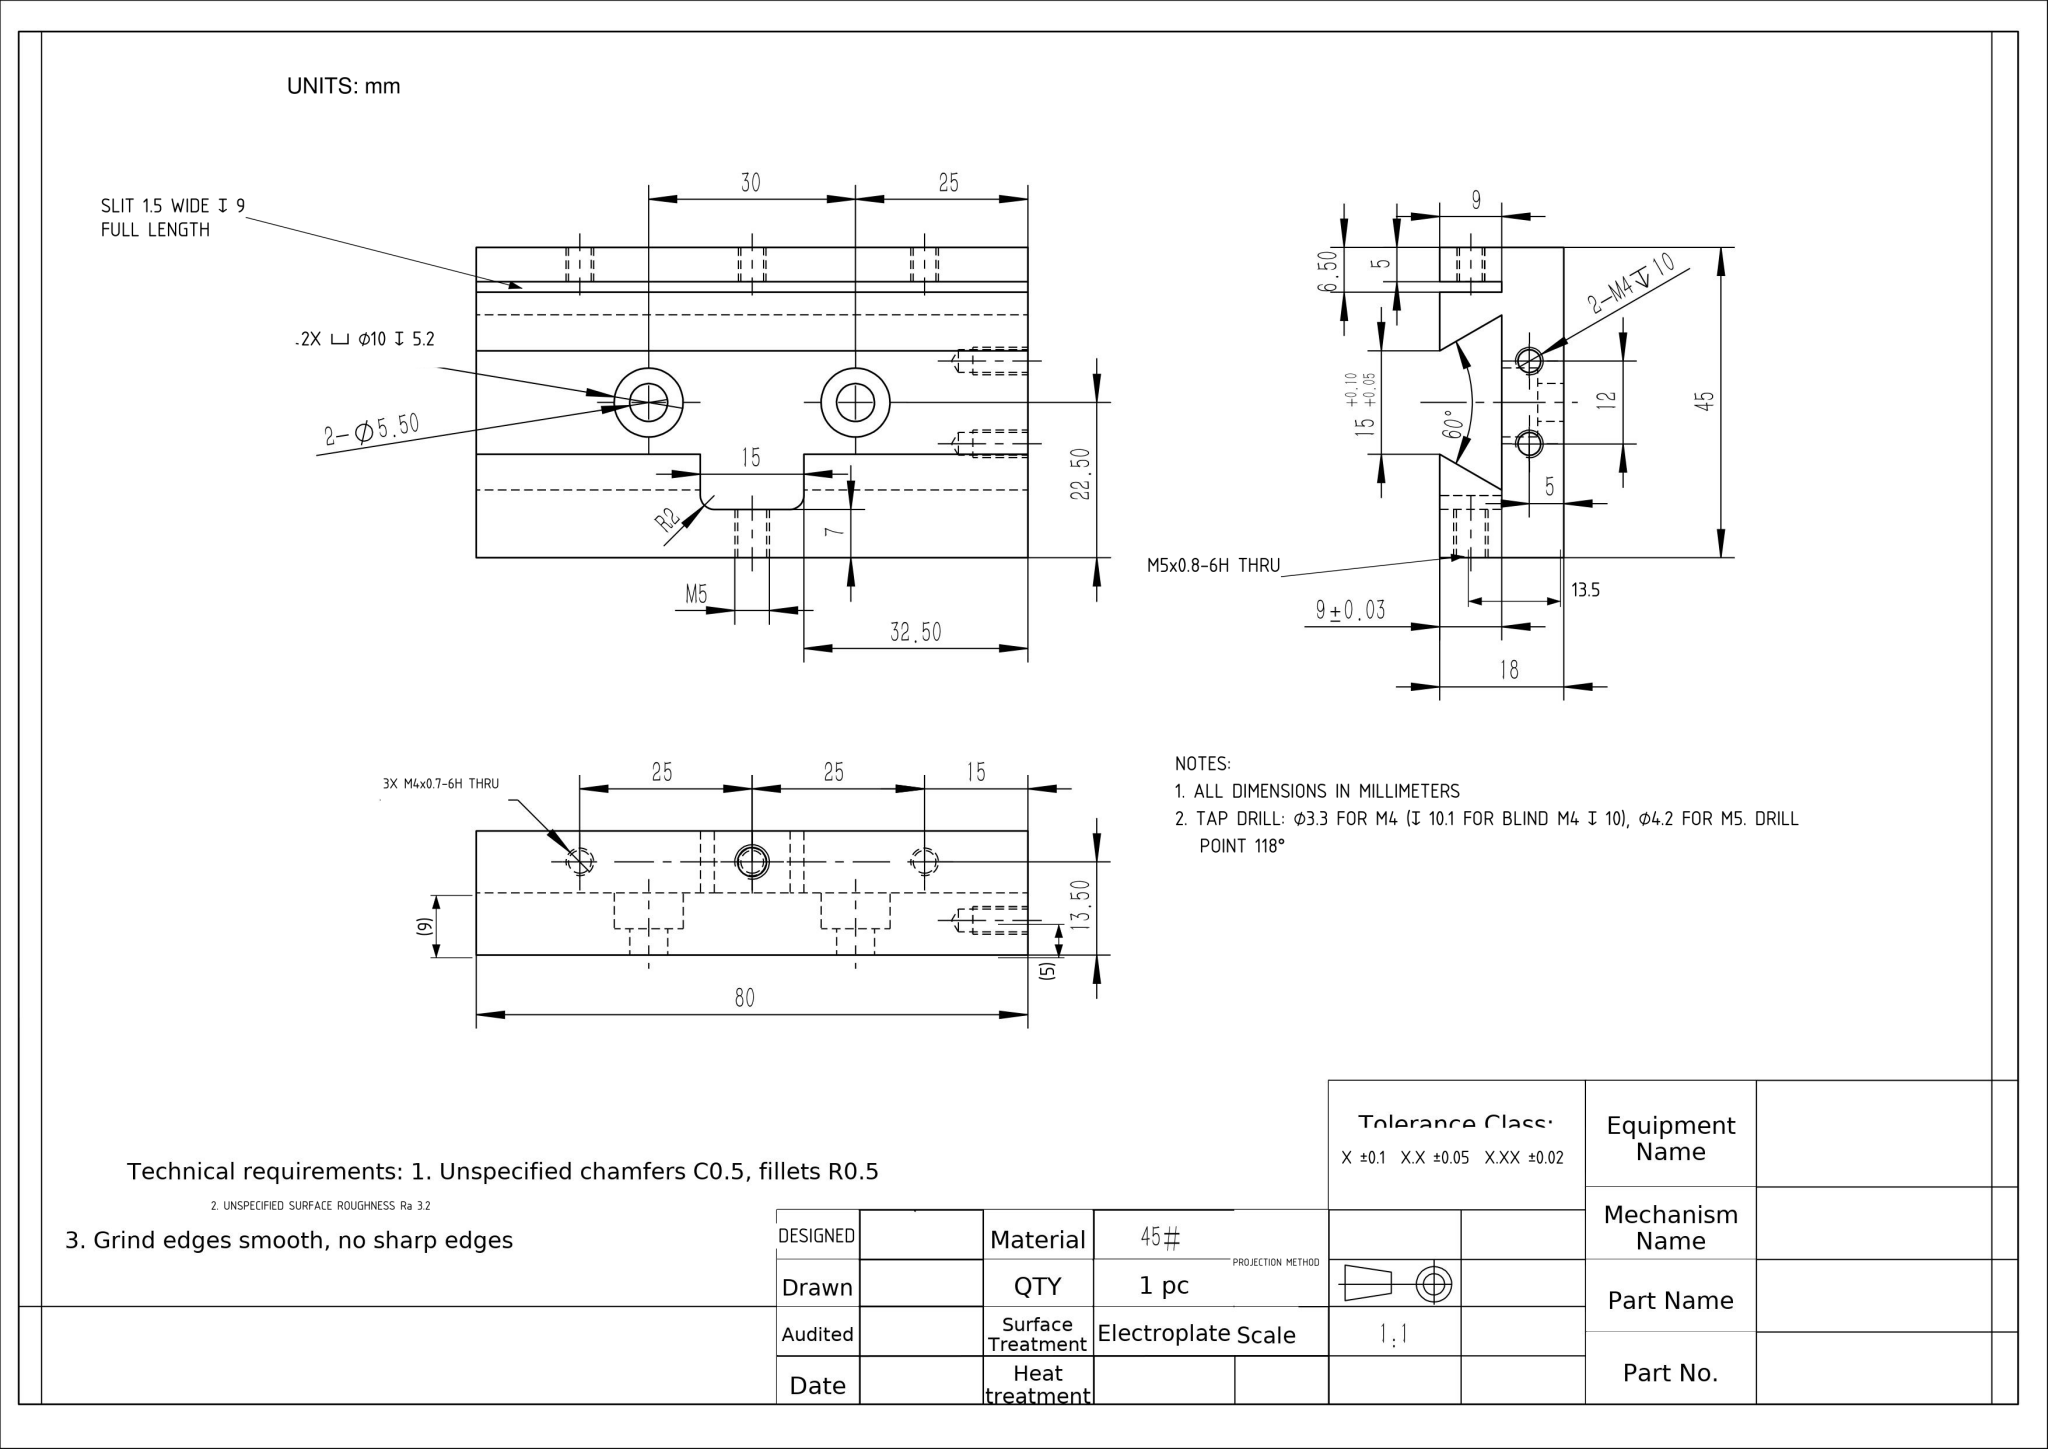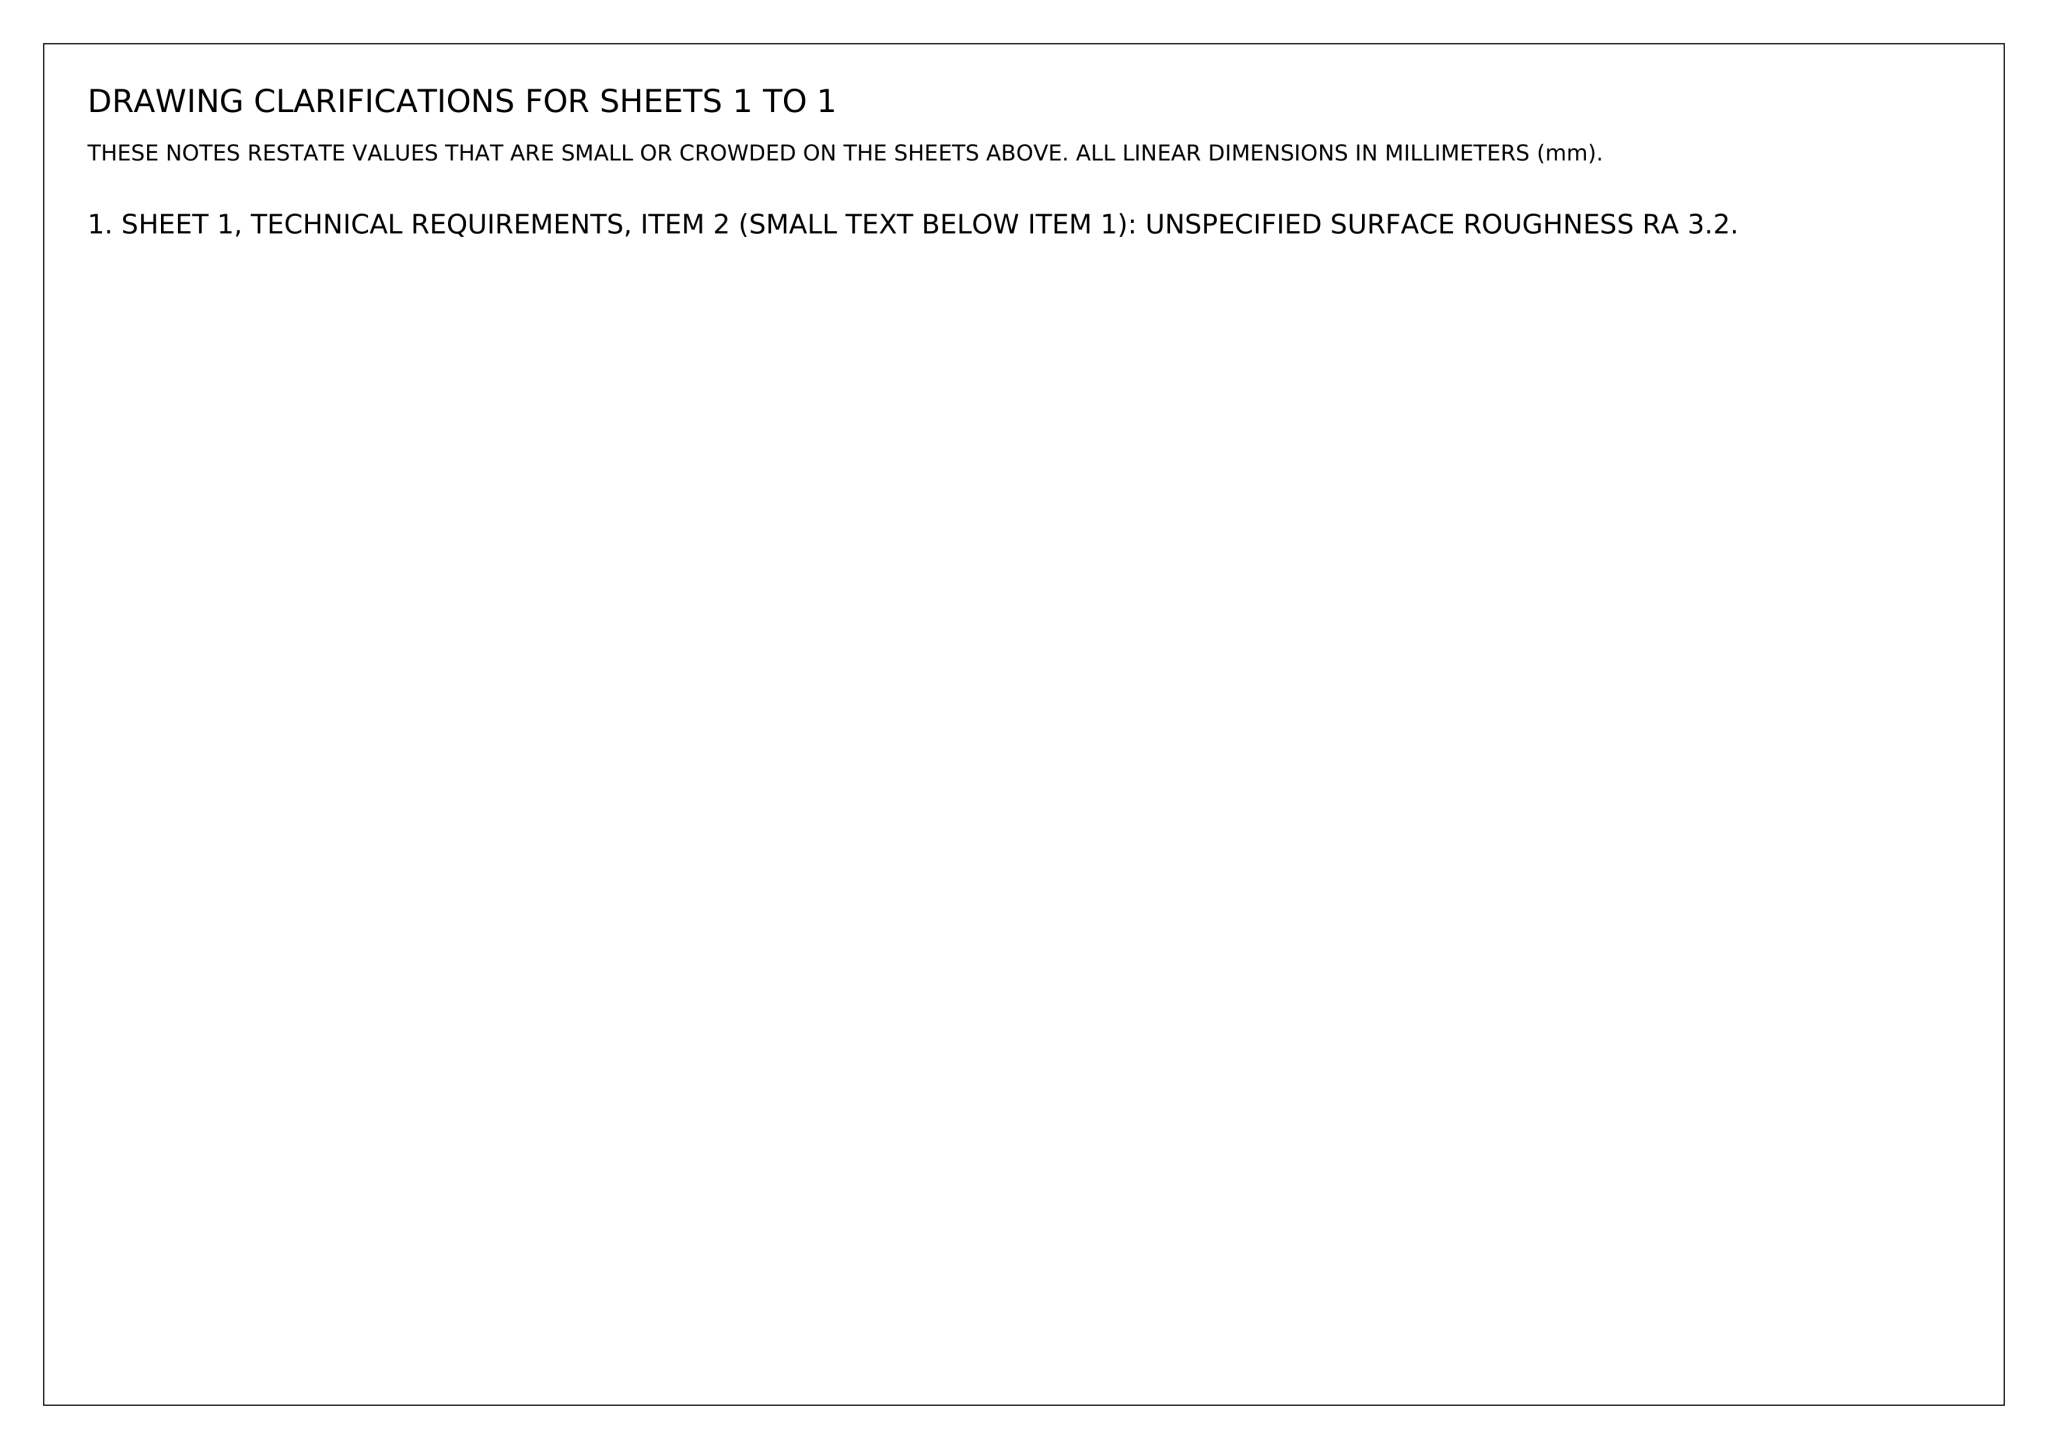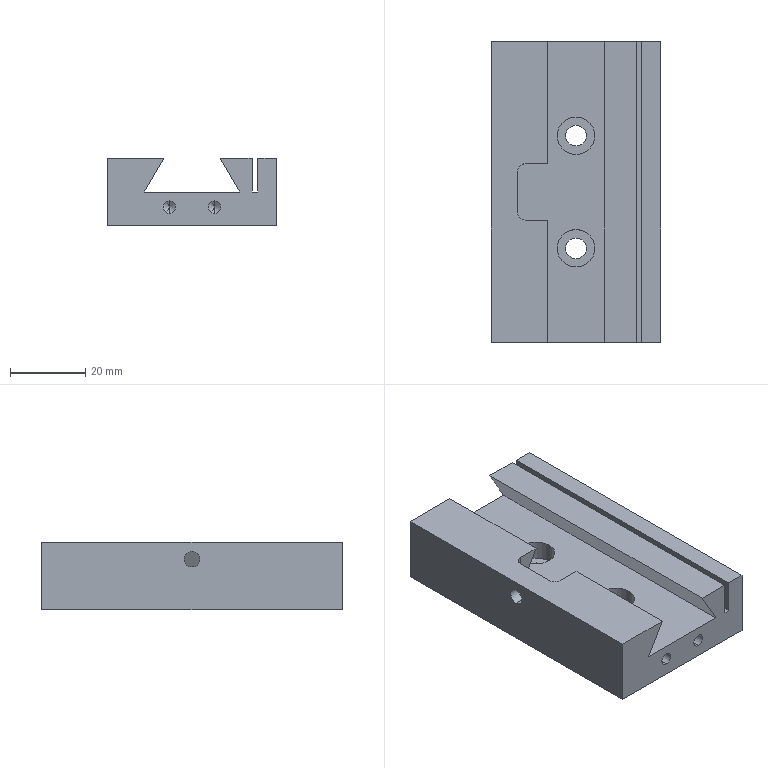Part | NX | mm | 1 solid | 46 faces | box 45 x 80 x 18 mm | volume 47064 mm3 | cylinder 22 | plane 20 | cone 4 | commonest cylinder face diameters 3.3 x10 10 x4 5.5 x4 4.2 x2 4 x2